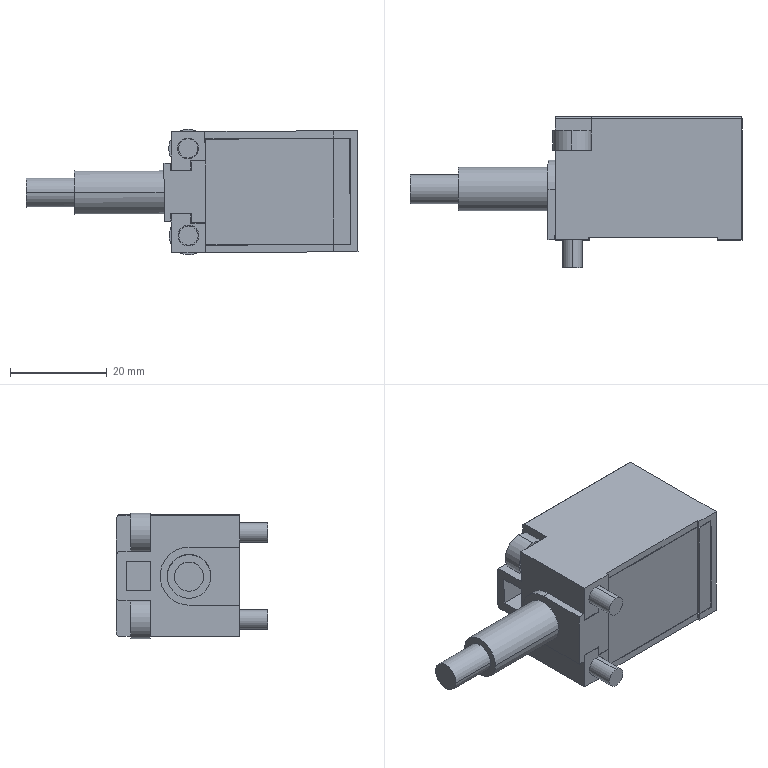Component | SolidWorks | TL_N5ME2-1 | 3 solids | 130 faces | volume 25383 mm3 | plane 95 | cylinder 35 | commonest cylinder face diameters 4 x6 12 x5 4.3 x4 17.6 x4 9.6 x4 8 x4 20 x2 9 x2